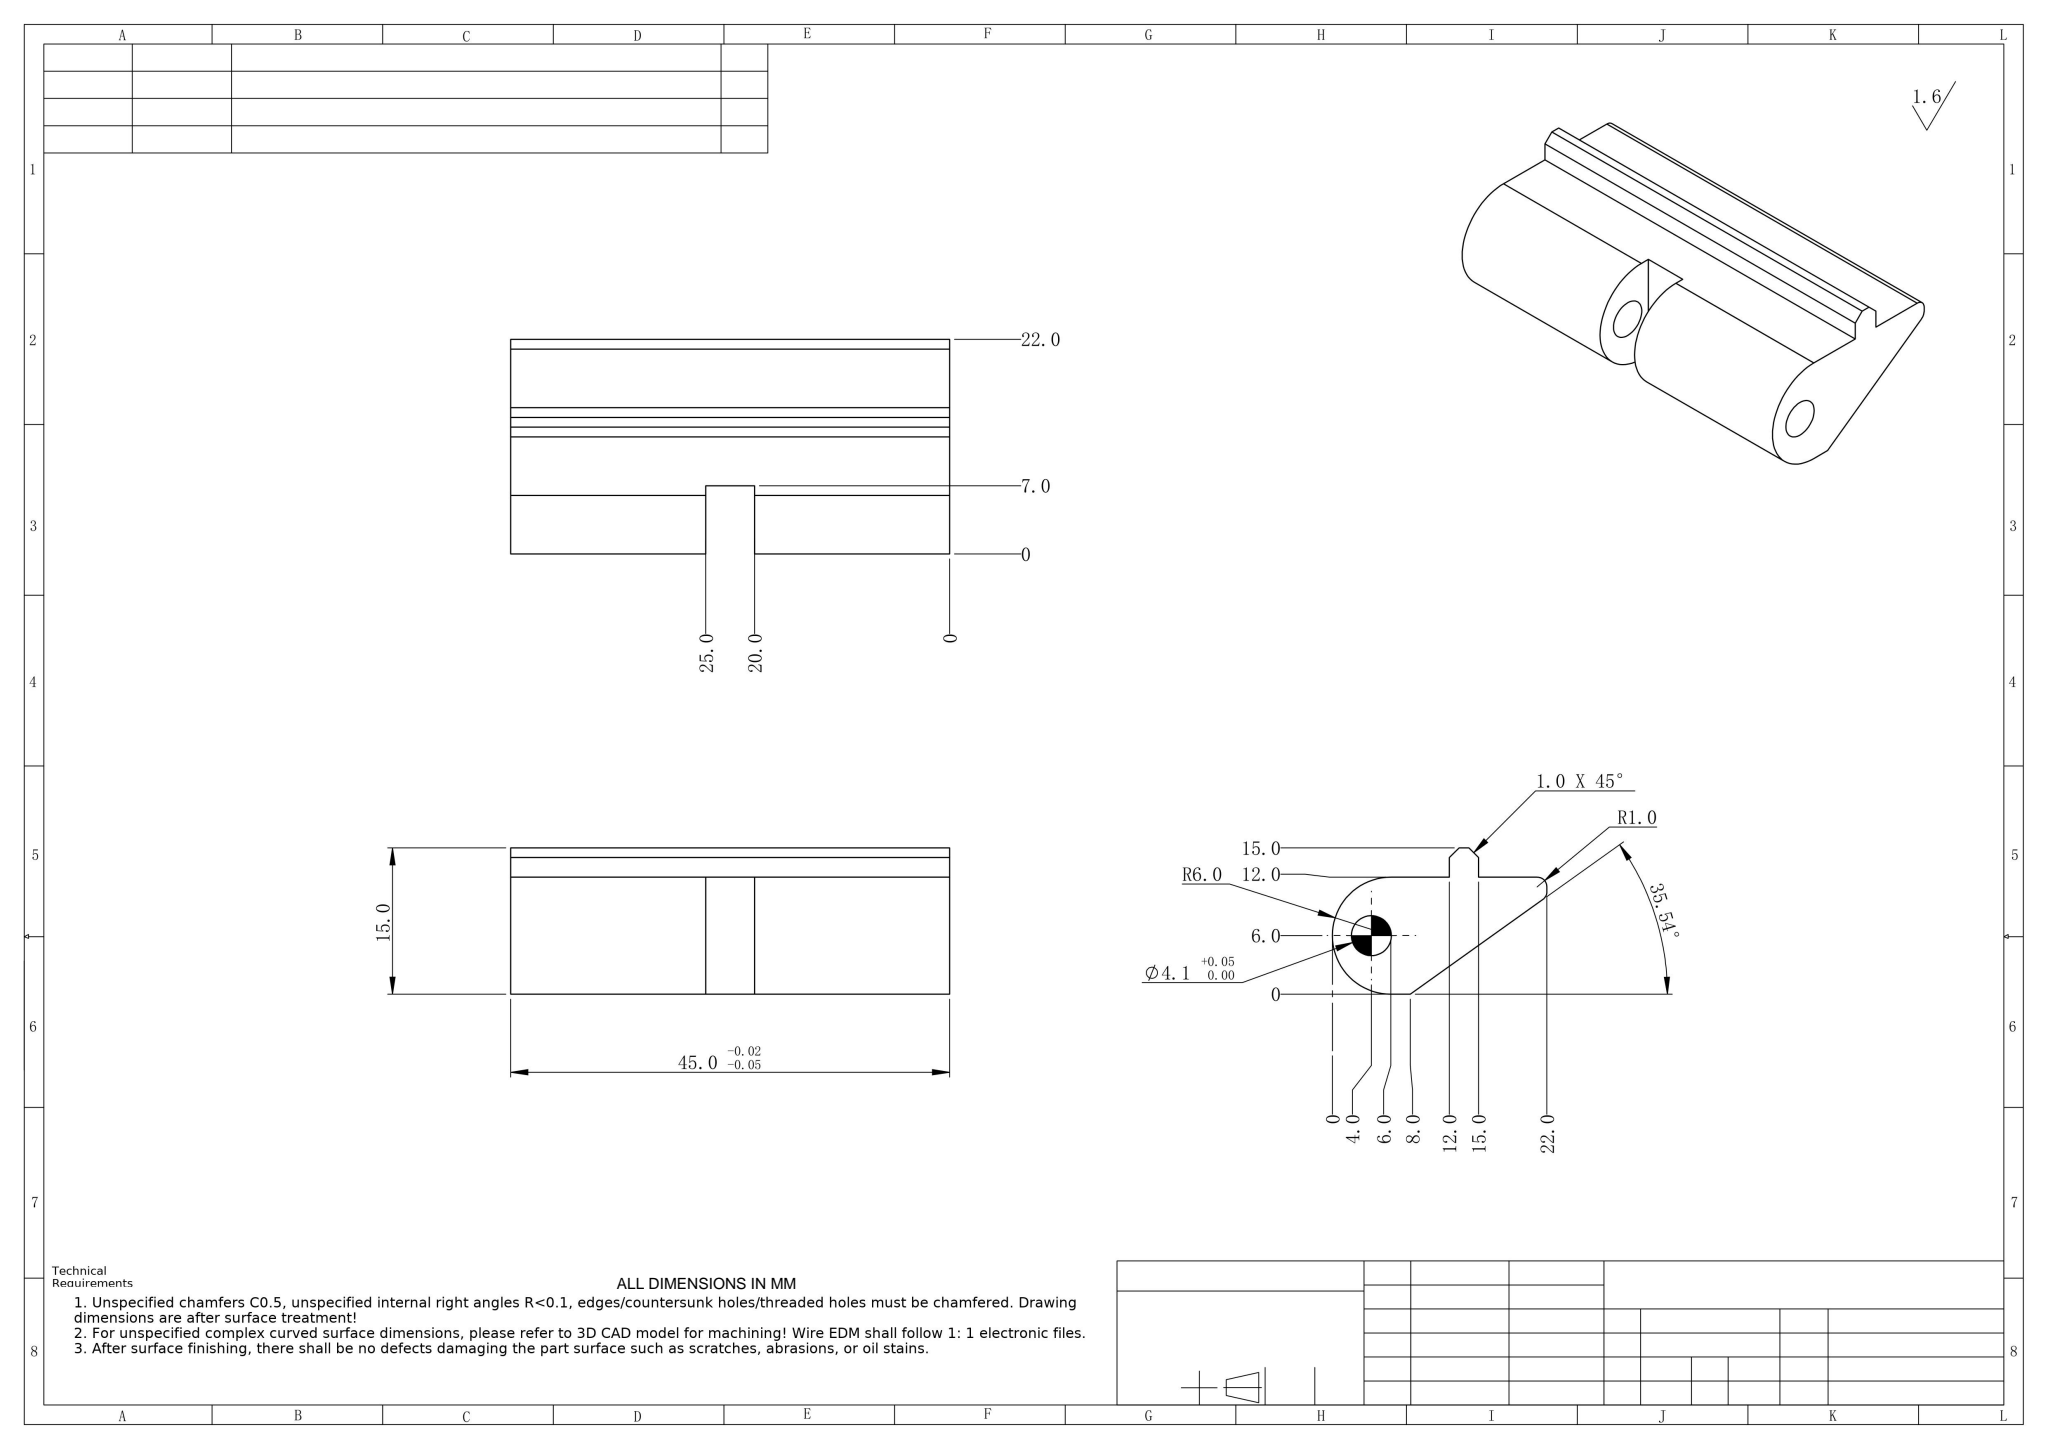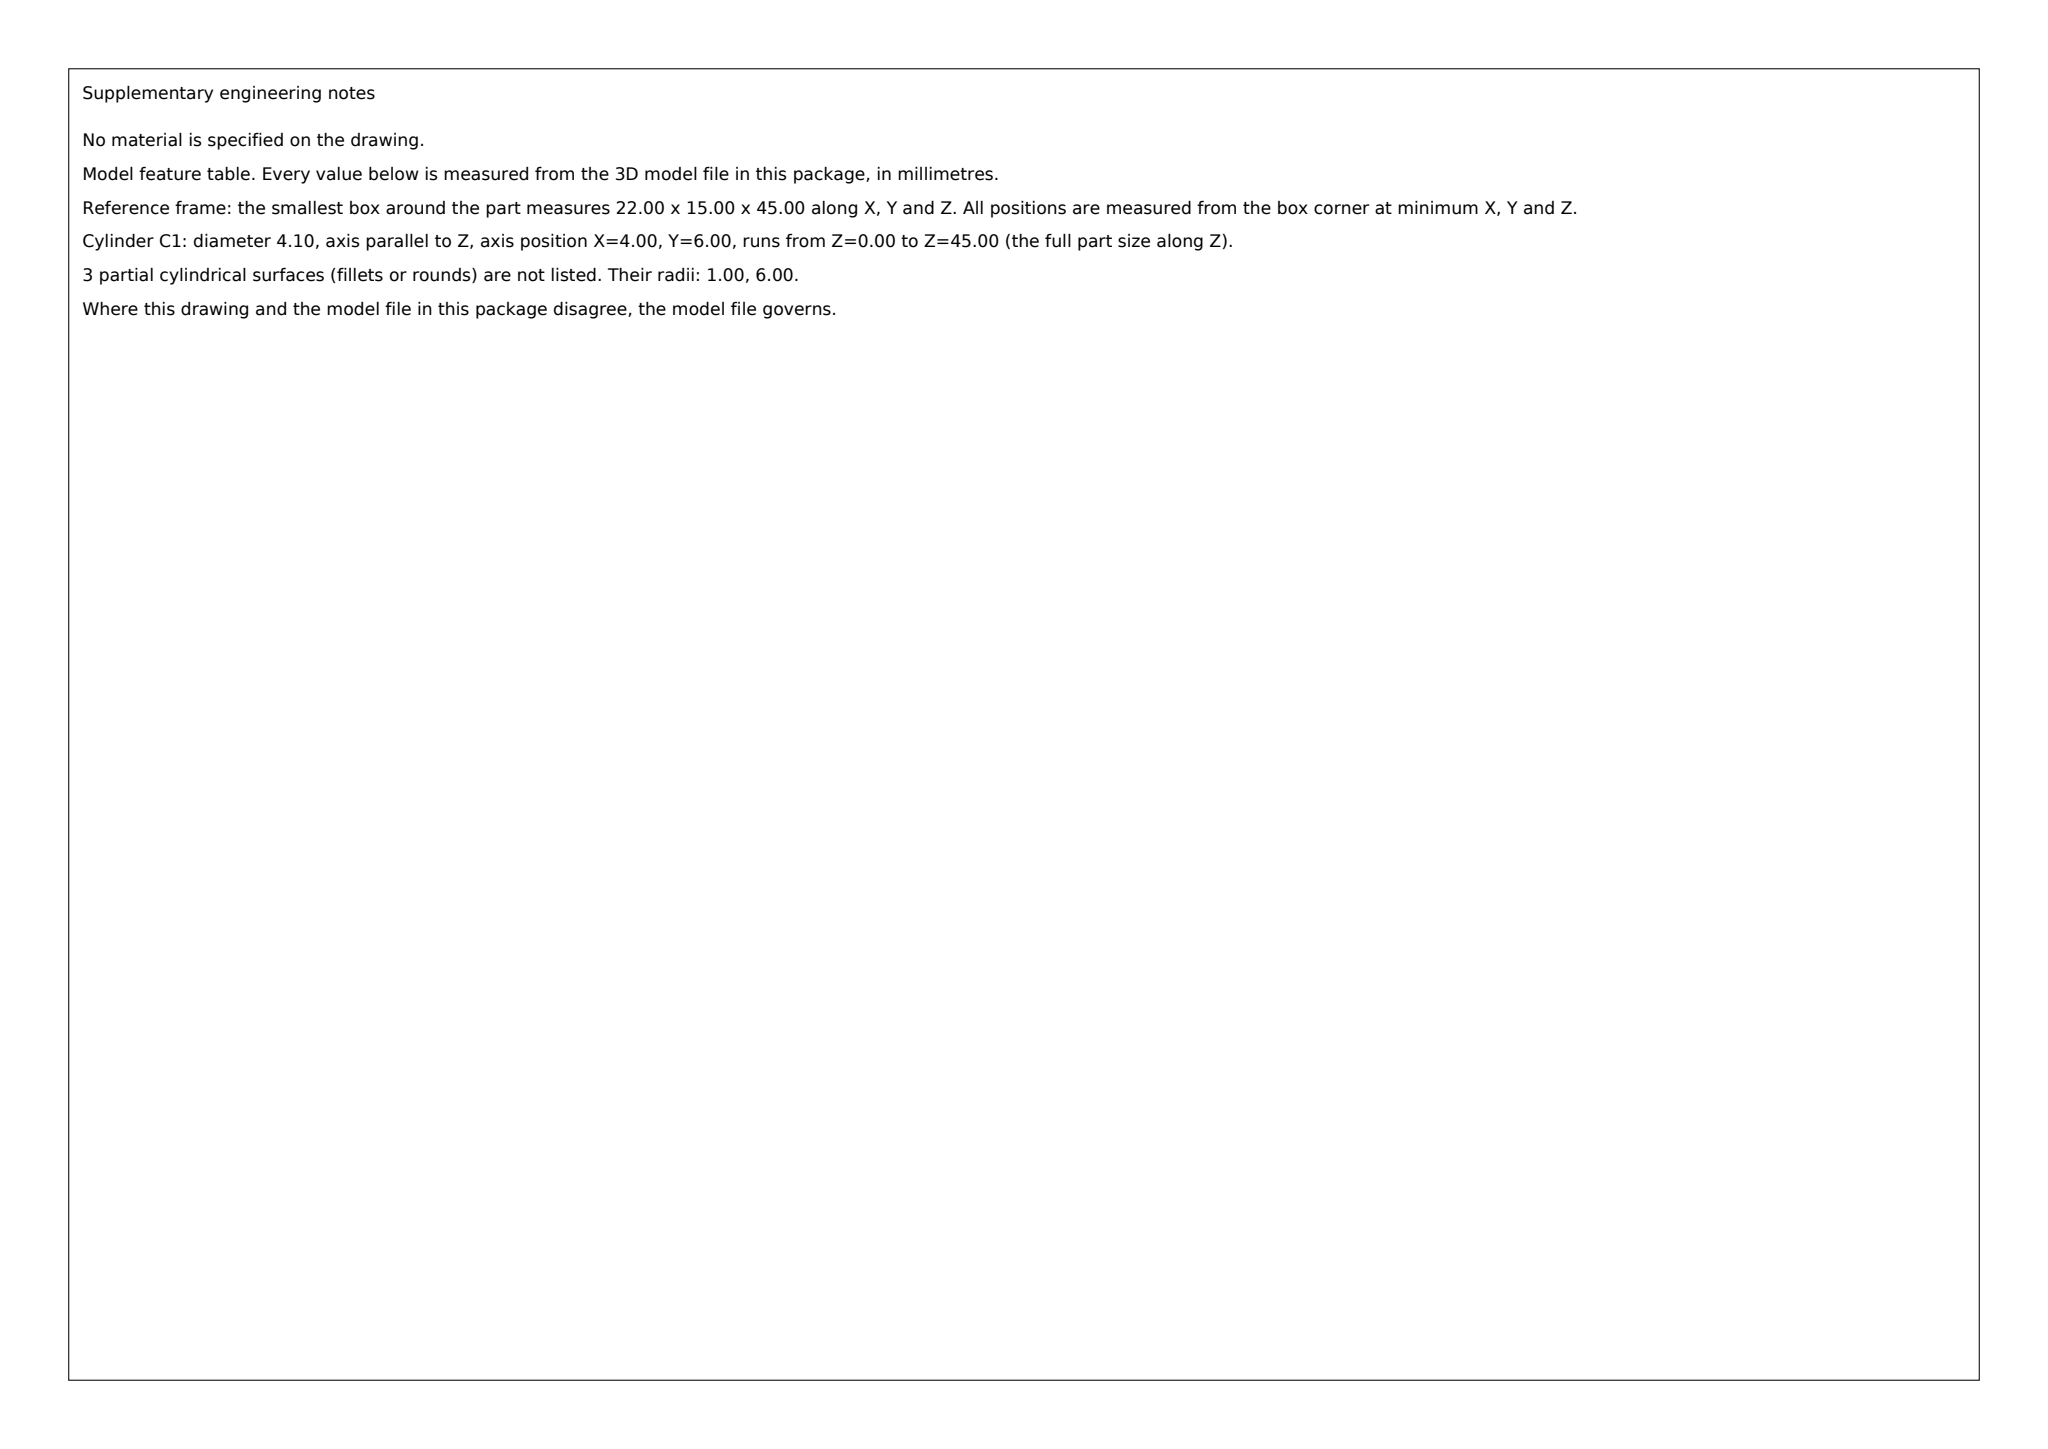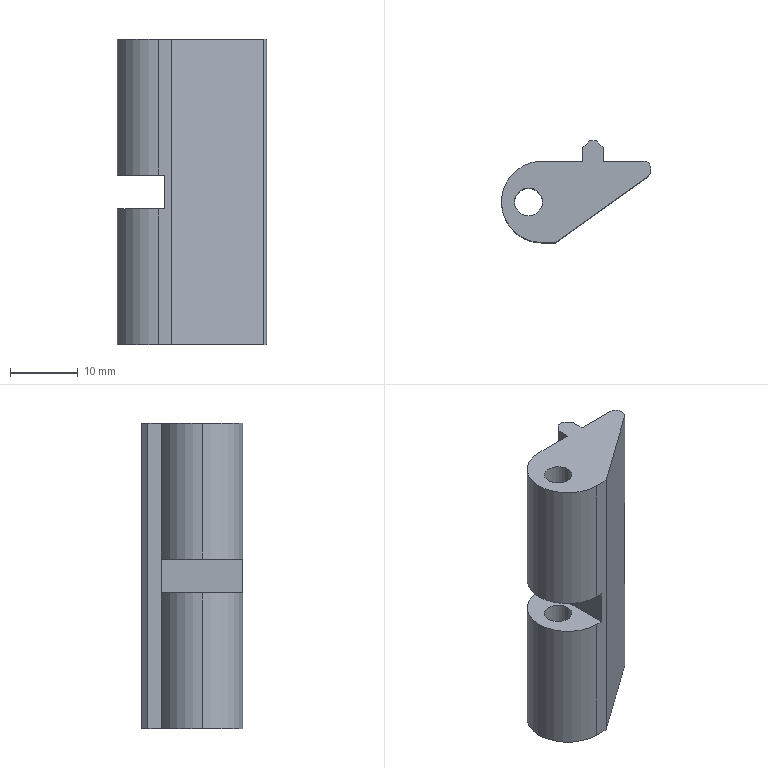Part | SolidWorks | mm | 1 solid | 25 faces | box 22 x 15 x 45 mm | volume 7512 mm3 | plane 15 | cylinder 10 | commonest cylinder face diameters 4.1 x4 12 x4 2 x2
build123d program:
from build123d import *

# Parameters (mm, degrees)
SKETCH1_R           = 2.05
BOSS_EXTRUDE1_DEPTH = 45
CHAMFER1_SIZE       = 1
SKETCH2_W           = 10
SKETCH2_H           = 5
CUT_EXTRUDE1_DEPTH  = 50.244
FILLET1_R           = 1


with BuildPart() as part:
    # Sketch1 → Boss-Extrude1 (new body)
    with BuildSketch(Plane.XY):
        with BuildLine():
            Line((9, 6), (16, 6))
            Line((16, 6), (16, 4))
            Line((16, 4), (2, -6))
            Line((2, -6), (0, -6))
            ThreePointArc((0, -6), (-6, 0), (0, 6))
            Line((0, 6), (6, 6))
            Line((6, 6), (6, 9))
            Line((6, 9), (9, 9))
            Line((9, 9), (9, 6))
        make_face()
        with Locations(Location((-2, 0, 0), (0, 0, 180))):
            Circle(SKETCH1_R, mode=Mode.SUBTRACT)
    extrude(amount=BOSS_EXTRUDE1_DEPTH)

    # Chamfer1
    chamfer1_edges = [part.edges().sort_by_distance(p)[0] for p in [
        (6, 9, 22.5),
        (9, 9, 22.5),
    ]]
    chamfer(chamfer1_edges, length=CHAMFER1_SIZE)

    # Sketch2 → Cut-Extrude1 (cut, through all)
    with BuildSketch(Plane(origin=(0, 6, 0), x_dir=(1, 0, 0), z_dir=(0, 1, 0))):
        with Locations((-4, -22.5)):
            Rectangle(SKETCH2_W, SKETCH2_H)
    extrude(amount=-CUT_EXTRUDE1_DEPTH, mode=Mode.SUBTRACT)

    # Fillet1
    fillet1_edges = [part.edges().sort_by_distance(p)[0] for p in [
        (16, 6, 22.5),
        (16, 4, 22.5),
    ]]
    fillet(fillet1_edges, radius=FILLET1_R)


solid = part.part
STEP:
#1=CARTESIAN_POINT('',(0.05,0.,20.));
#2=VERTEX_POINT('',#1);
#3=CARTESIAN_POINT('',(-4.05,0.,20.));
#4=VERTEX_POINT('',#3);
#5=CARTESIAN_POINT('',(-2.,0.,20.));
#6=DIRECTION('',(0.,0.,-1.));
#7=DIRECTION('',(-1.,0.,0.));
#8=AXIS2_PLACEMENT_3D('',#5,#6,#7);
#9=CIRCLE('',#8,2.05);
#10=EDGE_CURVE('',#2,#4,#9,.T.);
#11=ORIENTED_EDGE('',*,*,#10,.F.);
#12=CARTESIAN_POINT('',(0.05,0.,0.));
#13=VERTEX_POINT('',#12);
#14=CARTESIAN_POINT('',(0.05,0.,45.));
#15=DIRECTION('',(0.,0.,-1.));
#16=VECTOR('',#15,1000.);
#17=LINE('',#14,#16);
#18=EDGE_CURVE('',#2,#13,#17,.T.);
#19=ORIENTED_EDGE('',*,*,#18,.T.);
#20=CARTESIAN_POINT('',(-4.05,0.,0.));
#21=VERTEX_POINT('',#20);
#22=CARTESIAN_POINT('',(-2.,0.,0.));
#23=DIRECTION('',(0.,0.,1.));
#24=DIRECTION('',(1.,0.,0.));
#25=AXIS2_PLACEMENT_3D('',#22,#23,#24);
#26=CIRCLE('',#25,2.05);
#27=EDGE_CURVE('',#21,#13,#26,.T.);
#28=ORIENTED_EDGE('',*,*,#27,.F.);
#29=CARTESIAN_POINT('',(-4.05,0.,45.));
#30=DIRECTION('',(0.,0.,-1.));
#31=VECTOR('',#30,1000.);
#32=LINE('',#29,#31);
#33=EDGE_CURVE('',#4,#21,#32,.T.);
#34=ORIENTED_EDGE('',*,*,#33,.F.);
#35=EDGE_LOOP('',(#11,#19,#28,#34));
#36=FACE_OUTER_BOUND('',#35,.T.);
#37=CARTESIAN_POINT('',(-2.,0.,45.));
#38=DIRECTION('',(0.,0.,-1.));
#39=DIRECTION('',(-1.,0.,0.));
#40=AXIS2_PLACEMENT_3D('',#37,#38,#39);
#41=CYLINDRICAL_SURFACE('',#40,2.05);
#42=ADVANCED_FACE('',(#36),#41,.F.);
#43=CARTESIAN_POINT('',(0.,-6.,20.));
#44=VERTEX_POINT('',#43);
#45=CARTESIAN_POINT('',(-6.,-0.,20.));
#46=VERTEX_POINT('',#45);
#47=CARTESIAN_POINT('',(0.,-0.,20.));
#48=DIRECTION('',(0.,0.,-1.));
#49=DIRECTION('',(-1.,0.,0.));
#50=AXIS2_PLACEMENT_3D('',#47,#48,#49);
#51=CIRCLE('',#50,6.);
#52=EDGE_CURVE('',#44,#46,#51,.T.);
#53=ORIENTED_EDGE('',*,*,#52,.T.);
#54=CARTESIAN_POINT('',(-6.,-0.,0.));
#55=VERTEX_POINT('',#54);
#56=CARTESIAN_POINT('',(-6.,-0.,45.));
#57=DIRECTION('',(0.,0.,-1.));
#58=VECTOR('',#57,1000.);
#59=LINE('',#56,#58);
#60=EDGE_CURVE('',#46,#55,#59,.T.);
#61=ORIENTED_EDGE('',*,*,#60,.T.);
#62=CARTESIAN_POINT('',(0.,-6.,0.));
#63=VERTEX_POINT('',#62);
#64=CARTESIAN_POINT('',(0.,-0.,0.));
#65=DIRECTION('',(0.,0.,1.));
#66=DIRECTION('',(1.,0.,0.));
#67=AXIS2_PLACEMENT_3D('',#64,#65,#66);
#68=CIRCLE('',#67,6.);
#69=EDGE_CURVE('',#55,#63,#68,.T.);
#70=ORIENTED_EDGE('',*,*,#69,.T.);
#71=CARTESIAN_POINT('',(0.,-6.,45.));
#72=DIRECTION('',(0.,0.,-1.));
#73=VECTOR('',#72,1000.);
#74=LINE('',#71,#73);
#75=EDGE_CURVE('',#44,#63,#74,.T.);
#76=ORIENTED_EDGE('',*,*,#75,.F.);
#77=EDGE_LOOP('',(#53,#61,#70,#76));
#78=FACE_OUTER_BOUND('',#77,.T.);
#79=CARTESIAN_POINT('',(0.,-0.,45.));
#80=DIRECTION('',(0.,0.,-1.));
#81=DIRECTION('',(-1.,0.,0.));
#82=AXIS2_PLACEMENT_3D('',#79,#80,#81);
#83=CYLINDRICAL_SURFACE('',#82,6.);
#84=ADVANCED_FACE('',(#78),#83,.T.);
#85=CARTESIAN_POINT('',(-4.05,0.,45.));
#86=VERTEX_POINT('',#85);
#87=CARTESIAN_POINT('',(0.05,0.,45.));
#88=VERTEX_POINT('',#87);
#89=CARTESIAN_POINT('',(-2.,0.,45.));
#90=DIRECTION('',(0.,0.,1.));
#91=DIRECTION('',(1.,0.,0.));
#92=AXIS2_PLACEMENT_3D('',#89,#90,#91);
#93=CIRCLE('',#92,2.05);
#94=EDGE_CURVE('',#86,#88,#93,.T.);
#95=ORIENTED_EDGE('',*,*,#94,.T.);
#96=CARTESIAN_POINT('',(0.05,0.,25.));
#97=VERTEX_POINT('',#96);
#98=CARTESIAN_POINT('',(0.05,0.,45.));
#99=DIRECTION('',(0.,0.,-1.));
#100=VECTOR('',#99,1000.);
#101=LINE('',#98,#100);
#102=EDGE_CURVE('',#88,#97,#101,.T.);
#103=ORIENTED_EDGE('',*,*,#102,.T.);
#104=CARTESIAN_POINT('',(-4.05,0.,25.));
#105=VERTEX_POINT('',#104);
#106=CARTESIAN_POINT('',(-2.,0.,25.));
#107=DIRECTION('',(0.,0.,1.));
#108=DIRECTION('',(1.,0.,0.));
#109=AXIS2_PLACEMENT_3D('',#106,#107,#108);
#110=CIRCLE('',#109,2.05);
#111=EDGE_CURVE('',#105,#97,#110,.T.);
#112=ORIENTED_EDGE('',*,*,#111,.F.);
#113=CARTESIAN_POINT('',(-4.05,0.,45.));
#114=DIRECTION('',(0.,0.,-1.));
#115=VECTOR('',#114,1000.);
#116=LINE('',#113,#115);
#117=EDGE_CURVE('',#86,#105,#116,.T.);
#118=ORIENTED_EDGE('',*,*,#117,.F.);
#119=EDGE_LOOP('',(#95,#103,#112,#118));
#120=FACE_OUTER_BOUND('',#119,.T.);
#121=CARTESIAN_POINT('',(-2.,0.,45.));
#122=DIRECTION('',(0.,0.,-1.));
#123=DIRECTION('',(-1.,0.,0.));
#124=AXIS2_PLACEMENT_3D('',#121,#122,#123);
#125=CYLINDRICAL_SURFACE('',#124,2.05);
#126=ADVANCED_FACE('',(#120),#125,.F.);
#127=CARTESIAN_POINT('',(-6.,-0.,45.));
#128=VERTEX_POINT('',#127);
#129=CARTESIAN_POINT('',(0.,-6.,45.));
#130=VERTEX_POINT('',#129);
#131=CARTESIAN_POINT('',(0.,-0.,45.));
#132=DIRECTION('',(0.,0.,1.));
#133=DIRECTION('',(1.,0.,0.));
#134=AXIS2_PLACEMENT_3D('',#131,#132,#133);
#135=CIRCLE('',#134,6.);
#136=EDGE_CURVE('',#128,#130,#135,.T.);
#137=ORIENTED_EDGE('',*,*,#136,.F.);
#138=CARTESIAN_POINT('',(-6.,-0.,25.));
#139=VERTEX_POINT('',#138);
#140=CARTESIAN_POINT('',(-6.,-0.,45.));
#141=DIRECTION('',(0.,0.,-1.));
#142=VECTOR('',#141,1000.);
#143=LINE('',#140,#142);
#144=EDGE_CURVE('',#128,#139,#143,.T.);
#145=ORIENTED_EDGE('',*,*,#144,.T.);
#146=CARTESIAN_POINT('',(0.,-6.,25.));
#147=VERTEX_POINT('',#146);
#148=CARTESIAN_POINT('',(0.,-0.,25.));
#149=DIRECTION('',(0.,0.,1.));
#150=DIRECTION('',(1.,0.,-0.));
#151=AXIS2_PLACEMENT_3D('',#148,#149,#150);
#152=CIRCLE('',#151,6.);
#153=EDGE_CURVE('',#139,#147,#152,.T.);
#154=ORIENTED_EDGE('',*,*,#153,.T.);
#155=CARTESIAN_POINT('',(0.,-6.,45.));
#156=DIRECTION('',(0.,0.,-1.));
#157=VECTOR('',#156,1000.);
#158=LINE('',#155,#157);
#159=EDGE_CURVE('',#130,#147,#158,.T.);
#160=ORIENTED_EDGE('',*,*,#159,.F.);
#161=EDGE_LOOP('',(#137,#145,#154,#160));
#162=FACE_OUTER_BOUND('',#161,.T.);
#163=CARTESIAN_POINT('',(0.,-0.,45.));
#164=DIRECTION('',(0.,0.,-1.));
#165=DIRECTION('',(-1.,0.,0.));
#166=AXIS2_PLACEMENT_3D('',#163,#164,#165);
#167=CYLINDRICAL_SURFACE('',#166,6.);
#168=ADVANCED_FACE('',(#162),#167,.T.);
#169=ORIENTED_EDGE('',*,*,#144,.F.);
#170=CARTESIAN_POINT('',(0.,6.,45.));
#171=VERTEX_POINT('',#170);
#172=CARTESIAN_POINT('',(0.,-0.,45.));
#173=DIRECTION('',(0.,0.,1.));
#174=DIRECTION('',(1.,0.,0.));
#175=AXIS2_PLACEMENT_3D('',#172,#173,#174);
#176=CIRCLE('',#175,6.);
#177=EDGE_CURVE('',#171,#128,#176,.T.);
#178=ORIENTED_EDGE('',*,*,#177,.F.);
#179=CARTESIAN_POINT('',(0.,6.,25.));
#180=VERTEX_POINT('',#179);
#181=CARTESIAN_POINT('',(0.,6.,45.));
#182=DIRECTION('',(0.,0.,-1.));
#183=VECTOR('',#182,1000.);
#184=LINE('',#181,#183);
#185=EDGE_CURVE('',#171,#180,#184,.T.);
#186=ORIENTED_EDGE('',*,*,#185,.T.);
#187=CARTESIAN_POINT('',(0.,-0.,25.));
#188=DIRECTION('',(0.,0.,1.));
#189=DIRECTION('',(1.,0.,-0.));
#190=AXIS2_PLACEMENT_3D('',#187,#188,#189);
#191=CIRCLE('',#190,6.);
#192=EDGE_CURVE('',#180,#139,#191,.T.);
#193=ORIENTED_EDGE('',*,*,#192,.T.);
#194=EDGE_LOOP('',(#169,#178,#186,#193));
#195=FACE_OUTER_BOUND('',#194,.T.);
#196=CARTESIAN_POINT('',(0.,-0.,45.));
#197=DIRECTION('',(0.,0.,-1.));
#198=DIRECTION('',(-1.,0.,0.));
#199=AXIS2_PLACEMENT_3D('',#196,#197,#198);
#200=CYLINDRICAL_SURFACE('',#199,6.);
#201=ADVANCED_FACE('',(#195),#200,.T.);
#202=ORIENTED_EDGE('',*,*,#102,.F.);
#203=CARTESIAN_POINT('',(-2.,0.,45.));
#204=DIRECTION('',(0.,0.,1.));
#205=DIRECTION('',(1.,0.,0.));
#206=AXIS2_PLACEMENT_3D('',#203,#204,#205);
#207=CIRCLE('',#206,2.05);
#208=EDGE_CURVE('',#88,#86,#207,.T.);
#209=ORIENTED_EDGE('',*,*,#208,.T.);
#210=ORIENTED_EDGE('',*,*,#117,.T.);
#211=CARTESIAN_POINT('',(-2.,0.,25.));
#212=DIRECTION('',(0.,0.,1.));
#213=DIRECTION('',(1.,0.,0.));
#214=AXIS2_PLACEMENT_3D('',#211,#212,#213);
#215=CIRCLE('',#214,2.05);
#216=EDGE_CURVE('',#97,#105,#215,.T.);
#217=ORIENTED_EDGE('',*,*,#216,.F.);
#218=EDGE_LOOP('',(#202,#209,#210,#217));
#219=FACE_OUTER_BOUND('',#218,.T.);
#220=CARTESIAN_POINT('',(-2.,0.,45.));
#221=DIRECTION('',(0.,0.,-1.));
#222=DIRECTION('',(-1.,0.,0.));
#223=AXIS2_PLACEMENT_3D('',#220,#221,#222);
#224=CYLINDRICAL_SURFACE('',#223,2.05);
#225=ADVANCED_FACE('',(#219),#224,.F.);
#226=CARTESIAN_POINT('',(2.,-6.,45.));
#227=VERTEX_POINT('',#226);
#228=CARTESIAN_POINT('',(15.581,3.701,45.));
#229=VERTEX_POINT('',#228);
#230=CARTESIAN_POINT('',(16.,4.,45.));
#231=DIRECTION('',(0.8137,0.5812,0.));
#232=VECTOR('',#231,1000.);
#233=LINE('',#230,#232);
#234=EDGE_CURVE('',#227,#229,#233,.T.);
#235=ORIENTED_EDGE('',*,*,#234,.T.);
#236=CARTESIAN_POINT('',(16.,4.515,45.));
#237=VERTEX_POINT('',#236);
#238=CARTESIAN_POINT('',(15.,4.515,45.));
#239=DIRECTION('',(0.,0.,1.));
#240=DIRECTION('',(1.,0.,0.));
#241=AXIS2_PLACEMENT_3D('',#238,#239,#240);
#242=CIRCLE('',#241,1.);
#243=EDGE_CURVE('',#229,#237,#242,.T.);
#244=ORIENTED_EDGE('',*,*,#243,.T.);
#245=CARTESIAN_POINT('',(16.,5.,45.));
#246=VERTEX_POINT('',#245);
#247=CARTESIAN_POINT('',(16.,6.,45.));
#248=DIRECTION('',(0.,1.,0.));
#249=VECTOR('',#248,1000.);
#250=LINE('',#247,#249);
#251=EDGE_CURVE('',#237,#246,#250,.T.);
#252=ORIENTED_EDGE('',*,*,#251,.T.);
#253=CARTESIAN_POINT('',(15.,6.,45.));
#254=VERTEX_POINT('',#253);
#255=CARTESIAN_POINT('',(15.,5.,45.));
#256=DIRECTION('',(0.,0.,1.));
#257=DIRECTION('',(1.,0.,0.));
#258=AXIS2_PLACEMENT_3D('',#255,#256,#257);
#259=CIRCLE('',#258,1.);
#260=EDGE_CURVE('',#246,#254,#259,.T.);
#261=ORIENTED_EDGE('',*,*,#260,.T.);
#262=CARTESIAN_POINT('',(9.,6.,45.));
#263=VERTEX_POINT('',#262);
#264=CARTESIAN_POINT('',(9.,6.,45.));
#265=DIRECTION('',(-1.,0.,0.));
#266=VECTOR('',#265,1000.);
#267=LINE('',#264,#266);
#268=EDGE_CURVE('',#254,#263,#267,.T.);
#269=ORIENTED_EDGE('',*,*,#268,.T.);
#270=CARTESIAN_POINT('',(9.,8.,45.));
#271=VERTEX_POINT('',#270);
#272=CARTESIAN_POINT('',(9.,9.,45.));
#273=DIRECTION('',(0.,1.,0.));
#274=VECTOR('',#273,1000.);
#275=LINE('',#272,#274);
#276=EDGE_CURVE('',#263,#271,#275,.T.);
#277=ORIENTED_EDGE('',*,*,#276,.T.);
#278=CARTESIAN_POINT('',(8.,9.,45.));
#279=VERTEX_POINT('',#278);
#280=CARTESIAN_POINT('',(8.5,8.5,45.));
#281=DIRECTION('',(-0.7071,0.7071,0.));
#282=VECTOR('',#281,1000.);
#283=LINE('',#280,#282);
#284=EDGE_CURVE('',#271,#279,#283,.T.);
#285=ORIENTED_EDGE('',*,*,#284,.T.);
#286=CARTESIAN_POINT('',(7.,9.,45.));
#287=VERTEX_POINT('',#286);
#288=CARTESIAN_POINT('',(6.,9.,45.));
#289=DIRECTION('',(-1.,0.,0.));
#290=VECTOR('',#289,1000.);
#291=LINE('',#288,#290);
#292=EDGE_CURVE('',#279,#287,#291,.T.);
#293=ORIENTED_EDGE('',*,*,#292,.T.);
#294=CARTESIAN_POINT('',(6.,8.,45.));
#295=VERTEX_POINT('',#294);
#296=CARTESIAN_POINT('',(-1.,1.,45.));
#297=DIRECTION('',(-0.7071,-0.7071,0.));
#298=VECTOR('',#297,1000.);
#299=LINE('',#296,#298);
#300=EDGE_CURVE('',#287,#295,#299,.T.);
#301=ORIENTED_EDGE('',*,*,#300,.T.);
#302=CARTESIAN_POINT('',(6.,6.,45.));
#303=VERTEX_POINT('',#302);
#304=CARTESIAN_POINT('',(6.,6.,45.));
#305=DIRECTION('',(0.,-1.,0.));
#306=VECTOR('',#305,1000.);
#307=LINE('',#304,#306);
#308=EDGE_CURVE('',#295,#303,#307,.T.);
#309=ORIENTED_EDGE('',*,*,#308,.T.);
#310=CARTESIAN_POINT('',(0.,6.,45.));
#311=DIRECTION('',(-1.,0.,0.));
#312=VECTOR('',#311,1000.);
#313=LINE('',#310,#312);
#314=EDGE_CURVE('',#303,#171,#313,.T.);
#315=ORIENTED_EDGE('',*,*,#314,.T.);
#316=ORIENTED_EDGE('',*,*,#177,.T.);
#317=ORIENTED_EDGE('',*,*,#136,.T.);
#318=CARTESIAN_POINT('',(2.,-6.,45.));
#319=DIRECTION('',(1.,-0.,0.));
#320=VECTOR('',#319,1000.);
#321=LINE('',#318,#320);
#322=EDGE_CURVE('',#130,#227,#321,.T.);
#323=ORIENTED_EDGE('',*,*,#322,.T.);
#324=EDGE_LOOP('',(#235,#244,#252,#261,#269,#277,#285,#293,#301,#309,#315,#316,#317,#323));
#325=FACE_OUTER_BOUND('',#324,.T.);
#326=ORIENTED_EDGE('',*,*,#94,.F.);
#327=ORIENTED_EDGE('',*,*,#208,.F.);
#328=EDGE_LOOP('',(#326,#327));
#329=FACE_BOUND('',#328,.T.);
#330=CARTESIAN_POINT('',(0.,-0.,45.));
#331=DIRECTION('',(0.,0.,1.));
#332=DIRECTION('',(1.,0.,0.));
#333=AXIS2_PLACEMENT_3D('',#330,#331,#332);
#334=PLANE('',#333);
#335=ADVANCED_FACE('',(#325,#329),#334,.T.);
#336=CARTESIAN_POINT('',(16.,4.515,0.));
#337=VERTEX_POINT('',#336);
#338=CARTESIAN_POINT('',(16.,5.,0.));
#339=VERTEX_POINT('',#338);
#340=CARTESIAN_POINT('',(16.,6.,0.));
#341=DIRECTION('',(0.,1.,0.));
#342=VECTOR('',#341,1000.);
#343=LINE('',#340,#342);
#344=EDGE_CURVE('',#337,#339,#343,.T.);
#345=ORIENTED_EDGE('',*,*,#344,.F.);
#346=CARTESIAN_POINT('',(15.581,3.701,0.));
#347=VERTEX_POINT('',#346);
#348=CARTESIAN_POINT('',(15.,4.515,0.));
#349=DIRECTION('',(0.,0.,-1.));
#350=DIRECTION('',(1.,0.,0.));
#351=AXIS2_PLACEMENT_3D('',#348,#349,#350);
#352=CIRCLE('',#351,1.);
#353=EDGE_CURVE('',#337,#347,#352,.T.);
#354=ORIENTED_EDGE('',*,*,#353,.T.);
#355=CARTESIAN_POINT('',(2.,-6.,0.));
#356=VERTEX_POINT('',#355);
#357=CARTESIAN_POINT('',(16.,4.,0.));
#358=DIRECTION('',(0.8137,0.5812,0.));
#359=VECTOR('',#358,1000.);
#360=LINE('',#357,#359);
#361=EDGE_CURVE('',#356,#347,#360,.T.);
#362=ORIENTED_EDGE('',*,*,#361,.F.);
#363=CARTESIAN_POINT('',(2.,-6.,0.));
#364=DIRECTION('',(1.,-0.,0.));
#365=VECTOR('',#364,1000.);
#366=LINE('',#363,#365);
#367=EDGE_CURVE('',#63,#356,#366,.T.);
#368=ORIENTED_EDGE('',*,*,#367,.F.);
#369=ORIENTED_EDGE('',*,*,#69,.F.);
#370=CARTESIAN_POINT('',(0.,6.,0.));
#371=VERTEX_POINT('',#370);
#372=CARTESIAN_POINT('',(0.,-0.,0.));
#373=DIRECTION('',(0.,0.,1.));
#374=DIRECTION('',(1.,0.,0.));
#375=AXIS2_PLACEMENT_3D('',#372,#373,#374);
#376=CIRCLE('',#375,6.);
#377=EDGE_CURVE('',#371,#55,#376,.T.);
#378=ORIENTED_EDGE('',*,*,#377,.F.);
#379=CARTESIAN_POINT('',(6.,6.,0.));
#380=VERTEX_POINT('',#379);
#381=CARTESIAN_POINT('',(0.,6.,0.));
#382=DIRECTION('',(-1.,0.,0.));
#383=VECTOR('',#382,1000.);
#384=LINE('',#381,#383);
#385=EDGE_CURVE('',#380,#371,#384,.T.);
#386=ORIENTED_EDGE('',*,*,#385,.F.);
#387=CARTESIAN_POINT('',(6.,8.,0.));
#388=VERTEX_POINT('',#387);
#389=CARTESIAN_POINT('',(6.,6.,0.));
#390=DIRECTION('',(0.,-1.,0.));
#391=VECTOR('',#390,1000.);
#392=LINE('',#389,#391);
#393=EDGE_CURVE('',#388,#380,#392,.T.);
#394=ORIENTED_EDGE('',*,*,#393,.F.);
#395=CARTESIAN_POINT('',(7.,9.,0.));
#396=VERTEX_POINT('',#395);
#397=CARTESIAN_POINT('',(6.,8.,0.));
#398=DIRECTION('',(0.7071,0.7071,0.));
#399=VECTOR('',#398,1000.);
#400=LINE('',#397,#399);
#401=EDGE_CURVE('',#388,#396,#400,.T.);
#402=ORIENTED_EDGE('',*,*,#401,.T.);
#403=CARTESIAN_POINT('',(8.,9.,0.));
#404=VERTEX_POINT('',#403);
#405=CARTESIAN_POINT('',(6.,9.,0.));
#406=DIRECTION('',(-1.,0.,0.));
#407=VECTOR('',#406,1000.);
#408=LINE('',#405,#407);
#409=EDGE_CURVE('',#404,#396,#408,.T.);
#410=ORIENTED_EDGE('',*,*,#409,.F.);
#411=CARTESIAN_POINT('',(9.,8.,0.));
#412=VERTEX_POINT('',#411);
#413=CARTESIAN_POINT('',(8.,9.,0.));
#414=DIRECTION('',(0.7071,-0.7071,0.));
#415=VECTOR('',#414,1000.);
#416=LINE('',#413,#415);
#417=EDGE_CURVE('',#404,#412,#416,.T.);
#418=ORIENTED_EDGE('',*,*,#417,.T.);
#419=CARTESIAN_POINT('',(9.,6.,0.));
#420=VERTEX_POINT('',#419);
#421=CARTESIAN_POINT('',(9.,9.,0.));
#422=DIRECTION('',(0.,1.,0.));
#423=VECTOR('',#422,1000.);
#424=LINE('',#421,#423);
#425=EDGE_CURVE('',#420,#412,#424,.T.);
#426=ORIENTED_EDGE('',*,*,#425,.F.);
#427=CARTESIAN_POINT('',(15.,6.,0.));
#428=VERTEX_POINT('',#427);
#429=CARTESIAN_POINT('',(9.,6.,0.));
#430=DIRECTION('',(-1.,0.,0.));
#431=VECTOR('',#430,1000.);
#432=LINE('',#429,#431);
#433=EDGE_CURVE('',#428,#420,#432,.T.);
#434=ORIENTED_EDGE('',*,*,#433,.F.);
#435=CARTESIAN_POINT('',(15.,5.,0.));
#436=DIRECTION('',(0.,0.,-1.));
#437=DIRECTION('',(1.,0.,0.));
#438=AXIS2_PLACEMENT_3D('',#435,#436,#437);
#439=CIRCLE('',#438,1.);
#440=EDGE_CURVE('',#428,#339,#439,.T.);
#441=ORIENTED_EDGE('',*,*,#440,.T.);
#442=EDGE_LOOP('',(#345,#354,#362,#368,#369,#378,#386,#394,#402,#410,#418,#426,#434,#441));
#443=FACE_OUTER_BOUND('',#442,.T.);
#444=ORIENTED_EDGE('',*,*,#27,.T.);
#445=CARTESIAN_POINT('',(-2.,0.,0.));
#446=DIRECTION('',(0.,0.,1.));
#447=DIRECTION('',(1.,0.,0.));
#448=AXIS2_PLACEMENT_3D('',#445,#446,#447);
#449=CIRCLE('',#448,2.05);
#450=EDGE_CURVE('',#13,#21,#449,.T.);
#451=ORIENTED_EDGE('',*,*,#450,.T.);
#452=EDGE_LOOP('',(#444,#451));
#453=FACE_BOUND('',#452,.T.);
#454=CARTESIAN_POINT('',(0.,-0.,0.));
#455=DIRECTION('',(0.,0.,1.));
#456=DIRECTION('',(1.,0.,0.));
#457=AXIS2_PLACEMENT_3D('',#454,#455,#456);
#458=PLANE('',#457);
#459=ADVANCED_FACE('',(#443,#453),#458,.F.);
#460=ORIENTED_EDGE('',*,*,#60,.F.);
#461=CARTESIAN_POINT('',(0.,6.,20.));
#462=VERTEX_POINT('',#461);
#463=CARTESIAN_POINT('',(0.,-0.,20.));
#464=DIRECTION('',(0.,0.,-1.));
#465=DIRECTION('',(-1.,0.,0.));
#466=AXIS2_PLACEMENT_3D('',#463,#464,#465);
#467=CIRCLE('',#466,6.);
#468=EDGE_CURVE('',#46,#462,#467,.T.);
#469=ORIENTED_EDGE('',*,*,#468,.T.);
#470=CARTESIAN_POINT('',(0.,6.,45.));
#471=DIRECTION('',(0.,0.,-1.));
#472=VECTOR('',#471,1000.);
#473=LINE('',#470,#472);
#474=EDGE_CURVE('',#462,#371,#473,.T.);
#475=ORIENTED_EDGE('',*,*,#474,.T.);
#476=ORIENTED_EDGE('',*,*,#377,.T.);
#477=EDGE_LOOP('',(#460,#469,#475,#476));
#478=FACE_OUTER_BOUND('',#477,.T.);
#479=CARTESIAN_POINT('',(0.,-0.,45.));
#480=DIRECTION('',(0.,0.,-1.));
#481=DIRECTION('',(-1.,0.,0.));
#482=AXIS2_PLACEMENT_3D('',#479,#480,#481);
#483=CYLINDRICAL_SURFACE('',#482,6.);
#484=ADVANCED_FACE('',(#478),#483,.T.);
#485=ORIENTED_EDGE('',*,*,#159,.T.);
#486=CARTESIAN_POINT('',(1.,-6.,25.));
#487=VERTEX_POINT('',#486);
#488=CARTESIAN_POINT('',(1.,-6.,25.));
#489=DIRECTION('',(1.,0.,-0.));
#490=VECTOR('',#489,1000.);
#491=LINE('',#488,#490);
#492=EDGE_CURVE('',#147,#487,#491,.T.);
#493=ORIENTED_EDGE('',*,*,#492,.T.);
#494=CARTESIAN_POINT('',(1.,-6.,20.));
#495=VERTEX_POINT('',#494);
#496=CARTESIAN_POINT('',(1.,-6.,20.));
#497=DIRECTION('',(-0.,0.,-1.));
#498=VECTOR('',#497,1000.);
#499=LINE('',#496,#498);
#500=EDGE_CURVE('',#487,#495,#499,.T.);
#501=ORIENTED_EDGE('',*,*,#500,.T.);
#502=CARTESIAN_POINT('',(1.,-6.,20.));
#503=DIRECTION('',(-1.,0.,0.));
#504=VECTOR('',#503,1000.);
#505=LINE('',#502,#504);
#506=EDGE_CURVE('',#495,#44,#505,.T.);
#507=ORIENTED_EDGE('',*,*,#506,.T.);
#508=ORIENTED_EDGE('',*,*,#75,.T.);
#509=ORIENTED_EDGE('',*,*,#367,.T.);
#510=CARTESIAN_POINT('',(2.,-6.,45.));
#511=DIRECTION('',(0.,0.,-1.));
#512=VECTOR('',#511,1000.);
#513=LINE('',#510,#512);
#514=EDGE_CURVE('',#227,#356,#513,.T.);
#515=ORIENTED_EDGE('',*,*,#514,.F.);
#516=ORIENTED_EDGE('',*,*,#322,.F.);
#517=EDGE_LOOP('',(#485,#493,#501,#507,#508,#509,#515,#516));
#518=FACE_OUTER_BOUND('',#517,.T.);
#519=CARTESIAN_POINT('',(2.,-6.,45.));
#520=DIRECTION('',(0.,1.,0.));
#521=DIRECTION('',(-1.,0.,0.));
#522=AXIS2_PLACEMENT_3D('',#519,#520,#521);
#523=PLANE('',#522);
#524=ADVANCED_FACE('',(#518),#523,.F.);
#525=ORIENTED_EDGE('',*,*,#361,.T.);
#526=CARTESIAN_POINT('',(15.581,3.701,45.));
#527=DIRECTION('',(0.,0.,1.));
#528=VECTOR('',#527,1000.);
#529=LINE('',#526,#528);
#530=EDGE_CURVE('',#347,#229,#529,.T.);
#531=ORIENTED_EDGE('',*,*,#530,.T.);
#532=ORIENTED_EDGE('',*,*,#234,.F.);
#533=ORIENTED_EDGE('',*,*,#514,.T.);
#534=EDGE_LOOP('',(#525,#531,#532,#533));
#535=FACE_OUTER_BOUND('',#534,.T.);
#536=CARTESIAN_POINT('',(16.,4.,45.));
#537=DIRECTION('',(-0.5812,0.8137,0.));
#538=DIRECTION('',(-0.8137,-0.5812,0.));
#539=AXIS2_PLACEMENT_3D('',#536,#537,#538);
#540=PLANE('',#539);
#541=ADVANCED_FACE('',(#535),#540,.F.);
#542=ORIENTED_EDGE('',*,*,#251,.F.);
#543=CARTESIAN_POINT('',(16.,4.515,45.));
#544=DIRECTION('',(0.,0.,-1.));
#545=VECTOR('',#544,1000.);
#546=LINE('',#543,#545);
#547=EDGE_CURVE('',#237,#337,#546,.T.);
#548=ORIENTED_EDGE('',*,*,#547,.T.);
#549=ORIENTED_EDGE('',*,*,#344,.T.);
#550=CARTESIAN_POINT('',(16.,5.,45.));
#551=DIRECTION('',(0.,0.,1.));
#552=VECTOR('',#551,1000.);
#553=LINE('',#550,#552);
#554=EDGE_CURVE('',#339,#246,#553,.T.);
#555=ORIENTED_EDGE('',*,*,#554,.T.);
#556=EDGE_LOOP('',(#542,#548,#549,#555));
#557=FACE_OUTER_BOUND('',#556,.T.);
#558=CARTESIAN_POINT('',(16.,6.,45.));
#559=DIRECTION('',(-1.,0.,0.));
#560=DIRECTION('',(0.,0.,1.));
#561=AXIS2_PLACEMENT_3D('',#558,#559,#560);
#562=PLANE('',#561);
#563=ADVANCED_FACE('',(#557),#562,.F.);
#564=ORIENTED_EDGE('',*,*,#268,.F.);
#565=CARTESIAN_POINT('',(15.,6.,45.));
#566=DIRECTION('',(0.,0.,-1.));
#567=VECTOR('',#566,1000.);
#568=LINE('',#565,#567);
#569=EDGE_CURVE('',#254,#428,#568,.T.);
#570=ORIENTED_EDGE('',*,*,#569,.T.);
#571=ORIENTED_EDGE('',*,*,#433,.T.);
#572=CARTESIAN_POINT('',(9.,6.,45.));
#573=DIRECTION('',(0.,0.,-1.));
#574=VECTOR('',#573,1000.);
#575=LINE('',#572,#574);
#576=EDGE_CURVE('',#263,#420,#575,.T.);
#577=ORIENTED_EDGE('',*,*,#576,.F.);
#578=EDGE_LOOP('',(#564,#570,#571,#577));
#579=FACE_OUTER_BOUND('',#578,.T.);
#580=CARTESIAN_POINT('',(9.,6.,45.));
#581=DIRECTION('',(0.,-1.,0.));
#582=DIRECTION('',(0.,0.,-1.));
#583=AXIS2_PLACEMENT_3D('',#580,#581,#582);
#584=PLANE('',#583);
#585=ADVANCED_FACE('',(#579),#584,.F.);
#586=ORIENTED_EDGE('',*,*,#425,.T.);
#587=CARTESIAN_POINT('',(9.,8.,45.));
#588=DIRECTION('',(0.,0.,1.));
#589=VECTOR('',#588,1000.);
#590=LINE('',#587,#589);
#591=EDGE_CURVE('',#412,#271,#590,.T.);
#592=ORIENTED_EDGE('',*,*,#591,.T.);
#593=ORIENTED_EDGE('',*,*,#276,.F.);
#594=ORIENTED_EDGE('',*,*,#576,.T.);
#595=EDGE_LOOP('',(#586,#592,#593,#594));
#596=FACE_OUTER_BOUND('',#595,.T.);
#597=CARTESIAN_POINT('',(9.,9.,45.));
#598=DIRECTION('',(-1.,0.,0.));
#599=DIRECTION('',(0.,0.,1.));
#600=AXIS2_PLACEMENT_3D('',#597,#598,#599);
#601=PLANE('',#600);
#602=ADVANCED_FACE('',(#596),#601,.F.);
#603=ORIENTED_EDGE('',*,*,#409,.T.);
#604=CARTESIAN_POINT('',(7.,9.,45.));
#605=DIRECTION('',(0.,0.,1.));
#606=VECTOR('',#605,1000.);
#607=LINE('',#604,#606);
#608=EDGE_CURVE('',#396,#287,#607,.T.);
#609=ORIENTED_EDGE('',*,*,#608,.T.);
#610=ORIENTED_EDGE('',*,*,#292,.F.);
#611=CARTESIAN_POINT('',(8.,9.,45.));
#612=DIRECTION('',(0.,0.,-1.));
#613=VECTOR('',#612,1000.);
#614=LINE('',#611,#613);
#615=EDGE_CURVE('',#279,#404,#614,.T.);
#616=ORIENTED_EDGE('',*,*,#615,.T.);
#617=EDGE_LOOP('',(#603,#609,#610,#616));
#618=FACE_OUTER_BOUND('',#617,.T.);
#619=CARTESIAN_POINT('',(6.,9.,45.));
#620=DIRECTION('',(0.,-1.,0.));
#621=DIRECTION('',(0.,0.,-1.));
#622=AXIS2_PLACEMENT_3D('',#619,#620,#621);
#623=PLANE('',#622);
#624=ADVANCED_FACE('',(#618),#623,.F.);
#625=ORIENTED_EDGE('',*,*,#308,.F.);
#626=CARTESIAN_POINT('',(6.,8.,45.));
#627=DIRECTION('',(0.,0.,-1.));
#628=VECTOR('',#627,1000.);
#629=LINE('',#626,#628);
#630=EDGE_CURVE('',#295,#388,#629,.T.);
#631=ORIENTED_EDGE('',*,*,#630,.T.);
#632=ORIENTED_EDGE('',*,*,#393,.T.);
#633=CARTESIAN_POINT('',(6.,6.,45.));
#634=DIRECTION('',(0.,0.,-1.));
#635=VECTOR('',#634,1000.);
#636=LINE('',#633,#635);
#637=EDGE_CURVE('',#303,#380,#636,.T.);
#638=ORIENTED_EDGE('',*,*,#637,.F.);
#639=EDGE_LOOP('',(#625,#631,#632,#638));
#640=FACE_OUTER_BOUND('',#639,.T.);
#641=CARTESIAN_POINT('',(6.,6.,45.));
#642=DIRECTION('',(1.,0.,0.));
#643=DIRECTION('',(0.,0.,-1.));
#644=AXIS2_PLACEMENT_3D('',#641,#642,#643);
#645=PLANE('',#644);
#646=ADVANCED_FACE('',(#640),#645,.F.);
#647=CARTESIAN_POINT('',(1.,6.,25.));
#648=VERTEX_POINT('',#647);
#649=CARTESIAN_POINT('',(1.,6.,20.));
#650=VERTEX_POINT('',#649);
#651=CARTESIAN_POINT('',(1.,6.,20.));
#652=DIRECTION('',(-0.,0.,-1.));
#653=VECTOR('',#652,1000.);
#654=LINE('',#651,#653);
#655=EDGE_CURVE('',#648,#650,#654,.T.);
#656=ORIENTED_EDGE('',*,*,#655,.F.);
#657=CARTESIAN_POINT('',(1.,6.,25.));
#658=DIRECTION('',(1.,0.,-0.));
#659=VECTOR('',#658,1000.);
#660=LINE('',#657,#659);
#661=EDGE_CURVE('',#180,#648,#660,.T.);
#662=ORIENTED_EDGE('',*,*,#661,.F.);
#663=ORIENTED_EDGE('',*,*,#185,.F.);
#664=ORIENTED_EDGE('',*,*,#314,.F.);
#665=ORIENTED_EDGE('',*,*,#637,.T.);
#666=ORIENTED_EDGE('',*,*,#385,.T.);
#667=ORIENTED_EDGE('',*,*,#474,.F.);
#668=CARTESIAN_POINT('',(1.,6.,20.));
#669=DIRECTION('',(-1.,0.,0.));
#670=VECTOR('',#669,1000.);
#671=LINE('',#668,#670);
#672=EDGE_CURVE('',#650,#462,#671,.T.);
#673=ORIENTED_EDGE('',*,*,#672,.F.);
#674=EDGE_LOOP('',(#656,#662,#663,#664,#665,#666,#667,#673));
#675=FACE_OUTER_BOUND('',#674,.T.);
#676=CARTESIAN_POINT('',(0.,6.,45.));
#677=DIRECTION('',(0.,-1.,0.));
#678=DIRECTION('',(0.,0.,-1.));
#679=AXIS2_PLACEMENT_3D('',#676,#677,#678);
#680=PLANE('',#679);
#681=ADVANCED_FACE('',(#675),#680,.F.);
#682=ORIENTED_EDGE('',*,*,#18,.F.);
#683=CARTESIAN_POINT('',(-2.,0.,20.));
#684=DIRECTION('',(0.,0.,-1.));
#685=DIRECTION('',(-1.,0.,0.));
#686=AXIS2_PLACEMENT_3D('',#683,#684,#685);
#687=CIRCLE('',#686,2.05);
#688=EDGE_CURVE('',#4,#2,#687,.T.);
#689=ORIENTED_EDGE('',*,*,#688,.F.);
#690=ORIENTED_EDGE('',*,*,#33,.T.);
#691=ORIENTED_EDGE('',*,*,#450,.F.);
#692=EDGE_LOOP('',(#682,#689,#690,#691));
#693=FACE_OUTER_BOUND('',#692,.T.);
#694=CARTESIAN_POINT('',(-2.,0.,45.));
#695=DIRECTION('',(0.,0.,-1.));
#696=DIRECTION('',(-1.,0.,0.));
#697=AXIS2_PLACEMENT_3D('',#694,#695,#696);
#698=CYLINDRICAL_SURFACE('',#697,2.05);
#699=ADVANCED_FACE('',(#693),#698,.F.);
#700=ORIENTED_EDGE('',*,*,#300,.F.);
#701=ORIENTED_EDGE('',*,*,#608,.F.);
#702=ORIENTED_EDGE('',*,*,#401,.F.);
#703=ORIENTED_EDGE('',*,*,#630,.F.);
#704=EDGE_LOOP('',(#700,#701,#702,#703));
#705=FACE_OUTER_BOUND('',#704,.T.);
#706=CARTESIAN_POINT('',(6.,8.,45.));
#707=DIRECTION('',(0.7071,-0.7071,0.));
#708=DIRECTION('',(0.,0.,-1.));
#709=AXIS2_PLACEMENT_3D('',#706,#707,#708);
#710=PLANE('',#709);
#711=ADVANCED_FACE('',(#705),#710,.F.);
#712=ORIENTED_EDGE('',*,*,#284,.F.);
#713=ORIENTED_EDGE('',*,*,#591,.F.);
#714=ORIENTED_EDGE('',*,*,#417,.F.);
#715=ORIENTED_EDGE('',*,*,#615,.F.);
#716=EDGE_LOOP('',(#712,#713,#714,#715));
#717=FACE_OUTER_BOUND('',#716,.T.);
#718=CARTESIAN_POINT('',(8.,9.,45.));
#719=DIRECTION('',(-0.7071,-0.7071,0.));
#720=DIRECTION('',(0.,0.,-1.));
#721=AXIS2_PLACEMENT_3D('',#718,#719,#720);
#722=PLANE('',#721);
#723=ADVANCED_FACE('',(#717),#722,.F.);
#724=ORIENTED_EDGE('',*,*,#111,.T.);
#725=ORIENTED_EDGE('',*,*,#216,.T.);
#726=EDGE_LOOP('',(#724,#725));
#727=FACE_BOUND('',#726,.T.);
#728=ORIENTED_EDGE('',*,*,#661,.T.);
#729=CARTESIAN_POINT('',(1.,-6.,25.));
#730=DIRECTION('',(0.,1.,0.));
#731=VECTOR('',#730,1000.);
#732=LINE('',#729,#731);
#733=EDGE_CURVE('',#487,#648,#732,.T.);
#734=ORIENTED_EDGE('',*,*,#733,.F.);
#735=ORIENTED_EDGE('',*,*,#492,.F.);
#736=ORIENTED_EDGE('',*,*,#153,.F.);
#737=ORIENTED_EDGE('',*,*,#192,.F.);
#738=EDGE_LOOP('',(#728,#734,#735,#736,#737));
#739=FACE_OUTER_BOUND('',#738,.T.);
#740=CARTESIAN_POINT('',(1.,-6.,25.));
#741=DIRECTION('',(0.,0.,1.));
#742=DIRECTION('',(1.,0.,-0.));
#743=AXIS2_PLACEMENT_3D('',#740,#741,#742);
#744=PLANE('',#743);
#745=ADVANCED_FACE('',(#727,#739),#744,.F.);
#746=ORIENTED_EDGE('',*,*,#688,.T.);
#747=ORIENTED_EDGE('',*,*,#10,.T.);
#748=EDGE_LOOP('',(#746,#747));
#749=FACE_BOUND('',#748,.T.);
#750=ORIENTED_EDGE('',*,*,#506,.F.);
#751=CARTESIAN_POINT('',(1.,-6.,20.));
#752=DIRECTION('',(0.,1.,0.));
#753=VECTOR('',#752,1000.);
#754=LINE('',#751,#753);
#755=EDGE_CURVE('',#495,#650,#754,.T.);
#756=ORIENTED_EDGE('',*,*,#755,.T.);
#757=ORIENTED_EDGE('',*,*,#672,.T.);
#758=ORIENTED_EDGE('',*,*,#468,.F.);
#759=ORIENTED_EDGE('',*,*,#52,.F.);
#760=EDGE_LOOP('',(#750,#756,#757,#758,#759));
#761=FACE_OUTER_BOUND('',#760,.T.);
#762=CARTESIAN_POINT('',(1.,-6.,20.));
#763=DIRECTION('',(0.,0.,-1.));
#764=DIRECTION('',(-1.,0.,0.));
#765=AXIS2_PLACEMENT_3D('',#762,#763,#764);
#766=PLANE('',#765);
#767=ADVANCED_FACE('',(#749,#761),#766,.F.);
#768=ORIENTED_EDGE('',*,*,#655,.T.);
#769=ORIENTED_EDGE('',*,*,#755,.F.);
#770=ORIENTED_EDGE('',*,*,#500,.F.);
#771=ORIENTED_EDGE('',*,*,#733,.T.);
#772=EDGE_LOOP('',(#768,#769,#770,#771));
#773=FACE_OUTER_BOUND('',#772,.T.);
#774=CARTESIAN_POINT('',(1.,-6.,20.));
#775=DIRECTION('',(1.,0.,-0.));
#776=DIRECTION('',(-0.,0.,-1.));
#777=AXIS2_PLACEMENT_3D('',#774,#775,#776);
#778=PLANE('',#777);
#779=ADVANCED_FACE('',(#773),#778,.F.);
#780=ORIENTED_EDGE('',*,*,#243,.F.);
#781=ORIENTED_EDGE('',*,*,#530,.F.);
#782=ORIENTED_EDGE('',*,*,#353,.F.);
#783=ORIENTED_EDGE('',*,*,#547,.F.);
#784=EDGE_LOOP('',(#780,#781,#782,#783));
#785=FACE_OUTER_BOUND('',#784,.T.);
#786=CARTESIAN_POINT('',(15.,4.515,45.));
#787=DIRECTION('',(0.,0.,-1.));
#788=DIRECTION('',(-1.,0.,0.));
#789=AXIS2_PLACEMENT_3D('',#786,#787,#788);
#790=CYLINDRICAL_SURFACE('',#789,1.);
#791=ADVANCED_FACE('',(#785),#790,.T.);
#792=ORIENTED_EDGE('',*,*,#260,.F.);
#793=ORIENTED_EDGE('',*,*,#554,.F.);
#794=ORIENTED_EDGE('',*,*,#440,.F.);
#795=ORIENTED_EDGE('',*,*,#569,.F.);
#796=EDGE_LOOP('',(#792,#793,#794,#795));
#797=FACE_OUTER_BOUND('',#796,.T.);
#798=CARTESIAN_POINT('',(15.,5.,45.));
#799=DIRECTION('',(0.,0.,-1.));
#800=DIRECTION('',(-1.,0.,0.));
#801=AXIS2_PLACEMENT_3D('',#798,#799,#800);
#802=CYLINDRICAL_SURFACE('',#801,1.);
#803=ADVANCED_FACE('',(#797),#802,.T.);
#804=CLOSED_SHELL('',(#42,#84,#126,#168,#201,#225,#335,#459,#484,#524,#541,#563,#585,#602,#624,#646,#681,#699,#711,#723,#745,#767,#779,#791,#803));
#805=MANIFOLD_SOLID_BREP('',#804);
#806=CARTESIAN_POINT('',(0.,0.,0.));
#807=DIRECTION('',(0.,0.,1.));
#808=DIRECTION('',(1.,0.,0.));
#809=AXIS2_PLACEMENT_3D('',#806,#807,#808);
#810=(LENGTH_UNIT()NAMED_UNIT(*)SI_UNIT(.MILLI.,.METRE.));
#811=UNCERTAINTY_MEASURE_WITH_UNIT(LENGTH_MEASURE(0.00001),#810,'','');
#812=(NAMED_UNIT(*)PLANE_ANGLE_UNIT()SI_UNIT($,.RADIAN.));
#813=(NAMED_UNIT(*)SI_UNIT($,.STERADIAN.)SOLID_ANGLE_UNIT());
#814=(GEOMETRIC_REPRESENTATION_CONTEXT(3)GLOBAL_UNCERTAINTY_ASSIGNED_CONTEXT((#811))GLOBAL_UNIT_ASSIGNED_CONTEXT((#810,#812,#813))REPRESENTATION_CONTEXT('',''));
#815=ADVANCED_BREP_SHAPE_REPRESENTATION('',(#805,#809),#814);